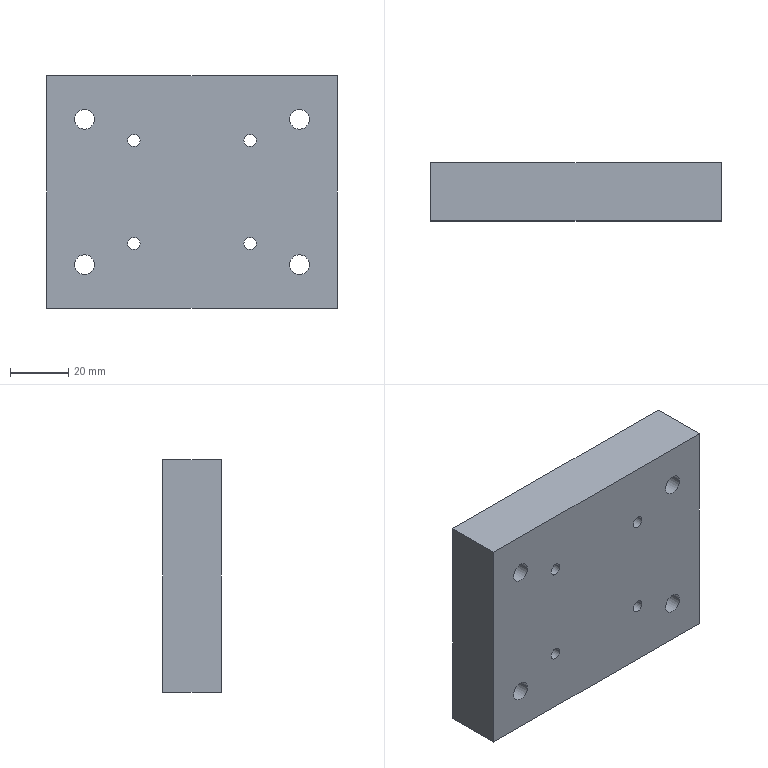Component | SolidWorks | RotaryCylinderBase-1 | 1 solid | 22 faces | box 100 x 20 x 80 mm | volume 155986 mm3 | cylinder 16 | plane 6 | commonest cylinder face diameters 6.8 x8 4.2 x8
build123d program:
from build123d import *

# Parameters (mm, degrees)
SKETCH2_W           = 100
SKETCH2_H           = 80
BOSS_EXTRUDE1_DEPTH = 20
M5_TAPPED_HOLE1_D   = 4.2
M8_TAPPED_HOLE1_D   = 6.8


with BuildPart() as part:
    # Sketch2 → Boss-Extrude1 (new body)
    with BuildSketch(Plane.XY):
        with Locations((233.487, -347.329)):
            Rectangle(SKETCH2_W, SKETCH2_H)
    extrude(amount=BOSS_EXTRUDE1_DEPTH)

    # M5 Tapped Hole1 (through all)
    with Locations(Plane.XY.offset(20)):
        with Locations((213.487, -365.079), (253.487, -365.079), (253.487, -329.579), (213.487, -329.579)):
            Hole(M5_TAPPED_HOLE1_D / 2)

    # M8 Tapped Hole1 (through all)
    with Locations(Plane(origin=(196.487, -322.329, 20), x_dir=(1, 0, 0), z_dir=(0, 0, 1))):
        with Locations((0, 0), (0, -50), (74, -50), (74, 0)):
            Hole(M8_TAPPED_HOLE1_D / 2)


solid = part.part

# Placed as in the assembly
solid = solid.moved(Location((-565.183, -127.651, 692.796), (90, 0, 0)))
STEP:
#1=COLOUR_RGB('',0.7922,0.8196,0.9333);
#2=FILL_AREA_STYLE_COLOUR('',#1);
#3=FILL_AREA_STYLE('',(#2));
#4=SURFACE_STYLE_FILL_AREA(#3);
#5=SURFACE_SIDE_STYLE('',(#4));
#6=SURFACE_STYLE_USAGE(.BOTH.,#5);
#7=PRESENTATION_STYLE_ASSIGNMENT((#6));
#8=CARTESIAN_POINT('',(-14.649,-5.813,12.617));
#9=VERTEX_POINT('',#8);
#10=CARTESIAN_POINT('',(-14.382,-5.813,12.617));
#11=VERTEX_POINT('',#10);
#12=CARTESIAN_POINT('',(-14.516,-5.813,12.617));
#13=DIRECTION('',(0.,1.,0.));
#14=DIRECTION('',(1.,0.,0.));
#15=AXIS2_PLACEMENT_3D('',#12,#13,#14);
#16=CIRCLE('',#15,0.1339);
#17=EDGE_CURVE('',#9,#11,#16,.T.);
#18=ORIENTED_EDGE('',*,*,#17,.F.);
#19=CARTESIAN_POINT('',(-14.649,-5.026,12.617));
#20=VERTEX_POINT('',#19);
#21=CARTESIAN_POINT('',(-14.649,-5.026,12.617));
#22=DIRECTION('',(0.,1.,0.));
#23=VECTOR('',#22,39.37);
#24=LINE('',#21,#23);
#25=EDGE_CURVE('',#9,#20,#24,.T.);
#26=ORIENTED_EDGE('',*,*,#25,.T.);
#27=CARTESIAN_POINT('',(-14.382,-5.026,12.617));
#28=VERTEX_POINT('',#27);
#29=CARTESIAN_POINT('',(-14.516,-5.026,12.617));
#30=DIRECTION('',(0.,1.,0.));
#31=DIRECTION('',(1.,0.,0.));
#32=AXIS2_PLACEMENT_3D('',#29,#30,#31);
#33=CIRCLE('',#32,0.1339);
#34=EDGE_CURVE('',#20,#28,#33,.T.);
#35=ORIENTED_EDGE('',*,*,#34,.T.);
#36=CARTESIAN_POINT('',(-14.382,-5.026,12.617));
#37=DIRECTION('',(0.,1.,0.));
#38=VECTOR('',#37,39.37);
#39=LINE('',#36,#38);
#40=EDGE_CURVE('',#11,#28,#39,.T.);
#41=ORIENTED_EDGE('',*,*,#40,.F.);
#42=EDGE_LOOP('',(#18,#26,#35,#41));
#43=FACE_OUTER_BOUND('',#42,.T.);
#44=CARTESIAN_POINT('',(-14.516,-5.026,12.617));
#45=DIRECTION('',(0.,1.,0.));
#46=DIRECTION('',(1.,0.,0.));
#47=AXIS2_PLACEMENT_3D('',#44,#45,#46);
#48=CYLINDRICAL_SURFACE('',#47,0.1339);
#49=ADVANCED_FACE('',(#43),#48,.F.);
#50=CARTESIAN_POINT('',(-14.649,-5.813,14.585));
#51=VERTEX_POINT('',#50);
#52=CARTESIAN_POINT('',(-14.382,-5.813,14.585));
#53=VERTEX_POINT('',#52);
#54=CARTESIAN_POINT('',(-14.516,-5.813,14.585));
#55=DIRECTION('',(0.,1.,0.));
#56=DIRECTION('',(1.,0.,0.));
#57=AXIS2_PLACEMENT_3D('',#54,#55,#56);
#58=CIRCLE('',#57,0.1339);
#59=EDGE_CURVE('',#51,#53,#58,.T.);
#60=ORIENTED_EDGE('',*,*,#59,.F.);
#61=CARTESIAN_POINT('',(-14.649,-5.026,14.585));
#62=VERTEX_POINT('',#61);
#63=CARTESIAN_POINT('',(-14.649,-5.026,14.585));
#64=DIRECTION('',(0.,1.,0.));
#65=VECTOR('',#64,39.37);
#66=LINE('',#63,#65);
#67=EDGE_CURVE('',#51,#62,#66,.T.);
#68=ORIENTED_EDGE('',*,*,#67,.T.);
#69=CARTESIAN_POINT('',(-14.382,-5.026,14.585));
#70=VERTEX_POINT('',#69);
#71=CARTESIAN_POINT('',(-14.516,-5.026,14.585));
#72=DIRECTION('',(0.,1.,0.));
#73=DIRECTION('',(1.,0.,0.));
#74=AXIS2_PLACEMENT_3D('',#71,#72,#73);
#75=CIRCLE('',#74,0.1339);
#76=EDGE_CURVE('',#62,#70,#75,.T.);
#77=ORIENTED_EDGE('',*,*,#76,.T.);
#78=CARTESIAN_POINT('',(-14.382,-5.026,14.585));
#79=DIRECTION('',(0.,1.,0.));
#80=VECTOR('',#79,39.37);
#81=LINE('',#78,#80);
#82=EDGE_CURVE('',#53,#70,#81,.T.);
#83=ORIENTED_EDGE('',*,*,#82,.F.);
#84=EDGE_LOOP('',(#60,#68,#77,#83));
#85=FACE_OUTER_BOUND('',#84,.T.);
#86=CARTESIAN_POINT('',(-14.516,-5.026,14.585));
#87=DIRECTION('',(0.,1.,0.));
#88=DIRECTION('',(1.,0.,0.));
#89=AXIS2_PLACEMENT_3D('',#86,#87,#88);
#90=CYLINDRICAL_SURFACE('',#89,0.1339);
#91=ADVANCED_FACE('',(#85),#90,.F.);
#92=CARTESIAN_POINT('',(-11.736,-5.813,14.585));
#93=VERTEX_POINT('',#92);
#94=CARTESIAN_POINT('',(-11.468,-5.813,14.585));
#95=VERTEX_POINT('',#94);
#96=CARTESIAN_POINT('',(-11.602,-5.813,14.585));
#97=DIRECTION('',(0.,1.,0.));
#98=DIRECTION('',(1.,0.,0.));
#99=AXIS2_PLACEMENT_3D('',#96,#97,#98);
#100=CIRCLE('',#99,0.1339);
#101=EDGE_CURVE('',#93,#95,#100,.T.);
#102=ORIENTED_EDGE('',*,*,#101,.F.);
#103=CARTESIAN_POINT('',(-11.736,-5.026,14.585));
#104=VERTEX_POINT('',#103);
#105=CARTESIAN_POINT('',(-11.736,-5.026,14.585));
#106=DIRECTION('',(0.,1.,0.));
#107=VECTOR('',#106,39.37);
#108=LINE('',#105,#107);
#109=EDGE_CURVE('',#93,#104,#108,.T.);
#110=ORIENTED_EDGE('',*,*,#109,.T.);
#111=CARTESIAN_POINT('',(-11.468,-5.026,14.585));
#112=VERTEX_POINT('',#111);
#113=CARTESIAN_POINT('',(-11.602,-5.026,14.585));
#114=DIRECTION('',(0.,1.,0.));
#115=DIRECTION('',(1.,0.,0.));
#116=AXIS2_PLACEMENT_3D('',#113,#114,#115);
#117=CIRCLE('',#116,0.1339);
#118=EDGE_CURVE('',#104,#112,#117,.T.);
#119=ORIENTED_EDGE('',*,*,#118,.T.);
#120=CARTESIAN_POINT('',(-11.468,-5.026,14.585));
#121=DIRECTION('',(0.,1.,0.));
#122=VECTOR('',#121,39.37);
#123=LINE('',#120,#122);
#124=EDGE_CURVE('',#95,#112,#123,.T.);
#125=ORIENTED_EDGE('',*,*,#124,.F.);
#126=EDGE_LOOP('',(#102,#110,#119,#125));
#127=FACE_OUTER_BOUND('',#126,.T.);
#128=CARTESIAN_POINT('',(-11.602,-5.026,14.585));
#129=DIRECTION('',(0.,1.,0.));
#130=DIRECTION('',(1.,0.,0.));
#131=AXIS2_PLACEMENT_3D('',#128,#129,#130);
#132=CYLINDRICAL_SURFACE('',#131,0.1339);
#133=ADVANCED_FACE('',(#127),#132,.F.);
#134=CARTESIAN_POINT('',(-11.736,-5.813,12.617));
#135=VERTEX_POINT('',#134);
#136=CARTESIAN_POINT('',(-11.468,-5.813,12.617));
#137=VERTEX_POINT('',#136);
#138=CARTESIAN_POINT('',(-11.602,-5.813,12.617));
#139=DIRECTION('',(0.,1.,0.));
#140=DIRECTION('',(1.,0.,0.));
#141=AXIS2_PLACEMENT_3D('',#138,#139,#140);
#142=CIRCLE('',#141,0.1339);
#143=EDGE_CURVE('',#135,#137,#142,.T.);
#144=ORIENTED_EDGE('',*,*,#143,.F.);
#145=CARTESIAN_POINT('',(-11.736,-5.026,12.617));
#146=VERTEX_POINT('',#145);
#147=CARTESIAN_POINT('',(-11.736,-5.026,12.617));
#148=DIRECTION('',(0.,1.,0.));
#149=VECTOR('',#148,39.37);
#150=LINE('',#147,#149);
#151=EDGE_CURVE('',#135,#146,#150,.T.);
#152=ORIENTED_EDGE('',*,*,#151,.T.);
#153=CARTESIAN_POINT('',(-11.468,-5.026,12.617));
#154=VERTEX_POINT('',#153);
#155=CARTESIAN_POINT('',(-11.602,-5.026,12.617));
#156=DIRECTION('',(0.,1.,0.));
#157=DIRECTION('',(1.,0.,0.));
#158=AXIS2_PLACEMENT_3D('',#155,#156,#157);
#159=CIRCLE('',#158,0.1339);
#160=EDGE_CURVE('',#146,#154,#159,.T.);
#161=ORIENTED_EDGE('',*,*,#160,.T.);
#162=CARTESIAN_POINT('',(-11.468,-5.026,12.617));
#163=DIRECTION('',(0.,1.,0.));
#164=VECTOR('',#163,39.37);
#165=LINE('',#162,#164);
#166=EDGE_CURVE('',#137,#154,#165,.T.);
#167=ORIENTED_EDGE('',*,*,#166,.F.);
#168=EDGE_LOOP('',(#144,#152,#161,#167));
#169=FACE_OUTER_BOUND('',#168,.T.);
#170=CARTESIAN_POINT('',(-11.602,-5.026,12.617));
#171=DIRECTION('',(0.,1.,0.));
#172=DIRECTION('',(1.,0.,0.));
#173=AXIS2_PLACEMENT_3D('',#170,#171,#172);
#174=CYLINDRICAL_SURFACE('',#173,0.1339);
#175=ADVANCED_FACE('',(#169),#174,.F.);
#176=CARTESIAN_POINT('',(-13.929,-5.813,14.3));
#177=VERTEX_POINT('',#176);
#178=CARTESIAN_POINT('',(-13.764,-5.813,14.3));
#179=VERTEX_POINT('',#178);
#180=CARTESIAN_POINT('',(-13.846,-5.813,14.3));
#181=DIRECTION('',(0.,1.,0.));
#182=DIRECTION('',(1.,0.,0.));
#183=AXIS2_PLACEMENT_3D('',#180,#181,#182);
#184=CIRCLE('',#183,0.08268);
#185=EDGE_CURVE('',#177,#179,#184,.T.);
#186=ORIENTED_EDGE('',*,*,#185,.F.);
#187=CARTESIAN_POINT('',(-13.929,-5.026,14.3));
#188=VERTEX_POINT('',#187);
#189=CARTESIAN_POINT('',(-13.929,-5.026,14.3));
#190=DIRECTION('',(0.,1.,0.));
#191=VECTOR('',#190,39.37);
#192=LINE('',#189,#191);
#193=EDGE_CURVE('',#177,#188,#192,.T.);
#194=ORIENTED_EDGE('',*,*,#193,.T.);
#195=CARTESIAN_POINT('',(-13.764,-5.026,14.3));
#196=VERTEX_POINT('',#195);
#197=CARTESIAN_POINT('',(-13.846,-5.026,14.3));
#198=DIRECTION('',(0.,1.,0.));
#199=DIRECTION('',(1.,0.,0.));
#200=AXIS2_PLACEMENT_3D('',#197,#198,#199);
#201=CIRCLE('',#200,0.08268);
#202=EDGE_CURVE('',#188,#196,#201,.T.);
#203=ORIENTED_EDGE('',*,*,#202,.T.);
#204=CARTESIAN_POINT('',(-13.764,-5.026,14.3));
#205=DIRECTION('',(0.,1.,0.));
#206=VECTOR('',#205,39.37);
#207=LINE('',#204,#206);
#208=EDGE_CURVE('',#179,#196,#207,.T.);
#209=ORIENTED_EDGE('',*,*,#208,.F.);
#210=EDGE_LOOP('',(#186,#194,#203,#209));
#211=FACE_OUTER_BOUND('',#210,.T.);
#212=CARTESIAN_POINT('',(-13.846,-5.026,14.3));
#213=DIRECTION('',(0.,1.,0.));
#214=DIRECTION('',(1.,0.,0.));
#215=AXIS2_PLACEMENT_3D('',#212,#213,#214);
#216=CYLINDRICAL_SURFACE('',#215,0.08268);
#217=ADVANCED_FACE('',(#211),#216,.F.);
#218=CARTESIAN_POINT('',(-12.354,-5.813,14.3));
#219=VERTEX_POINT('',#218);
#220=CARTESIAN_POINT('',(-12.189,-5.813,14.3));
#221=VERTEX_POINT('',#220);
#222=CARTESIAN_POINT('',(-12.271,-5.813,14.3));
#223=DIRECTION('',(0.,1.,0.));
#224=DIRECTION('',(1.,0.,0.));
#225=AXIS2_PLACEMENT_3D('',#222,#223,#224);
#226=CIRCLE('',#225,0.08268);
#227=EDGE_CURVE('',#219,#221,#226,.T.);
#228=ORIENTED_EDGE('',*,*,#227,.F.);
#229=CARTESIAN_POINT('',(-12.354,-5.026,14.3));
#230=VERTEX_POINT('',#229);
#231=CARTESIAN_POINT('',(-12.354,-5.026,14.3));
#232=DIRECTION('',(0.,1.,0.));
#233=VECTOR('',#232,39.37);
#234=LINE('',#231,#233);
#235=EDGE_CURVE('',#219,#230,#234,.T.);
#236=ORIENTED_EDGE('',*,*,#235,.T.);
#237=CARTESIAN_POINT('',(-12.189,-5.026,14.3));
#238=VERTEX_POINT('',#237);
#239=CARTESIAN_POINT('',(-12.271,-5.026,14.3));
#240=DIRECTION('',(0.,1.,0.));
#241=DIRECTION('',(1.,0.,0.));
#242=AXIS2_PLACEMENT_3D('',#239,#240,#241);
#243=CIRCLE('',#242,0.08268);
#244=EDGE_CURVE('',#230,#238,#243,.T.);
#245=ORIENTED_EDGE('',*,*,#244,.T.);
#246=CARTESIAN_POINT('',(-12.189,-5.026,14.3));
#247=DIRECTION('',(0.,1.,0.));
#248=VECTOR('',#247,39.37);
#249=LINE('',#246,#248);
#250=EDGE_CURVE('',#221,#238,#249,.T.);
#251=ORIENTED_EDGE('',*,*,#250,.F.);
#252=EDGE_LOOP('',(#228,#236,#245,#251));
#253=FACE_OUTER_BOUND('',#252,.T.);
#254=CARTESIAN_POINT('',(-12.271,-5.026,14.3));
#255=DIRECTION('',(0.,1.,0.));
#256=DIRECTION('',(1.,0.,0.));
#257=AXIS2_PLACEMENT_3D('',#254,#255,#256);
#258=CYLINDRICAL_SURFACE('',#257,0.08268);
#259=ADVANCED_FACE('',(#253),#258,.F.);
#260=CARTESIAN_POINT('',(-12.354,-5.813,12.902));
#261=VERTEX_POINT('',#260);
#262=CARTESIAN_POINT('',(-12.189,-5.813,12.902));
#263=VERTEX_POINT('',#262);
#264=CARTESIAN_POINT('',(-12.271,-5.813,12.902));
#265=DIRECTION('',(0.,1.,0.));
#266=DIRECTION('',(1.,0.,0.));
#267=AXIS2_PLACEMENT_3D('',#264,#265,#266);
#268=CIRCLE('',#267,0.08268);
#269=EDGE_CURVE('',#261,#263,#268,.T.);
#270=ORIENTED_EDGE('',*,*,#269,.F.);
#271=CARTESIAN_POINT('',(-12.354,-5.026,12.902));
#272=VERTEX_POINT('',#271);
#273=CARTESIAN_POINT('',(-12.354,-5.026,12.902));
#274=DIRECTION('',(0.,1.,0.));
#275=VECTOR('',#274,39.37);
#276=LINE('',#273,#275);
#277=EDGE_CURVE('',#261,#272,#276,.T.);
#278=ORIENTED_EDGE('',*,*,#277,.T.);
#279=CARTESIAN_POINT('',(-12.189,-5.026,12.902));
#280=VERTEX_POINT('',#279);
#281=CARTESIAN_POINT('',(-12.271,-5.026,12.902));
#282=DIRECTION('',(0.,1.,0.));
#283=DIRECTION('',(1.,0.,0.));
#284=AXIS2_PLACEMENT_3D('',#281,#282,#283);
#285=CIRCLE('',#284,0.08268);
#286=EDGE_CURVE('',#272,#280,#285,.T.);
#287=ORIENTED_EDGE('',*,*,#286,.T.);
#288=CARTESIAN_POINT('',(-12.189,-5.026,12.902));
#289=DIRECTION('',(0.,1.,0.));
#290=VECTOR('',#289,39.37);
#291=LINE('',#288,#290);
#292=EDGE_CURVE('',#263,#280,#291,.T.);
#293=ORIENTED_EDGE('',*,*,#292,.F.);
#294=EDGE_LOOP('',(#270,#278,#287,#293));
#295=FACE_OUTER_BOUND('',#294,.T.);
#296=CARTESIAN_POINT('',(-12.271,-5.026,12.902));
#297=DIRECTION('',(0.,1.,0.));
#298=DIRECTION('',(1.,0.,0.));
#299=AXIS2_PLACEMENT_3D('',#296,#297,#298);
#300=CYLINDRICAL_SURFACE('',#299,0.08268);
#301=ADVANCED_FACE('',(#295),#300,.F.);
#302=CARTESIAN_POINT('',(-13.929,-5.813,12.902));
#303=VERTEX_POINT('',#302);
#304=CARTESIAN_POINT('',(-13.764,-5.813,12.902));
#305=VERTEX_POINT('',#304);
#306=CARTESIAN_POINT('',(-13.846,-5.813,12.902));
#307=DIRECTION('',(0.,1.,0.));
#308=DIRECTION('',(1.,0.,0.));
#309=AXIS2_PLACEMENT_3D('',#306,#307,#308);
#310=CIRCLE('',#309,0.08268);
#311=EDGE_CURVE('',#303,#305,#310,.T.);
#312=ORIENTED_EDGE('',*,*,#311,.F.);
#313=CARTESIAN_POINT('',(-13.929,-5.026,12.902));
#314=VERTEX_POINT('',#313);
#315=CARTESIAN_POINT('',(-13.929,-5.026,12.902));
#316=DIRECTION('',(0.,1.,0.));
#317=VECTOR('',#316,39.37);
#318=LINE('',#315,#317);
#319=EDGE_CURVE('',#303,#314,#318,.T.);
#320=ORIENTED_EDGE('',*,*,#319,.T.);
#321=CARTESIAN_POINT('',(-13.764,-5.026,12.902));
#322=VERTEX_POINT('',#321);
#323=CARTESIAN_POINT('',(-13.846,-5.026,12.902));
#324=DIRECTION('',(0.,1.,0.));
#325=DIRECTION('',(1.,0.,0.));
#326=AXIS2_PLACEMENT_3D('',#323,#324,#325);
#327=CIRCLE('',#326,0.08268);
#328=EDGE_CURVE('',#314,#322,#327,.T.);
#329=ORIENTED_EDGE('',*,*,#328,.T.);
#330=CARTESIAN_POINT('',(-13.764,-5.026,12.902));
#331=DIRECTION('',(0.,1.,0.));
#332=VECTOR('',#331,39.37);
#333=LINE('',#330,#332);
#334=EDGE_CURVE('',#305,#322,#333,.T.);
#335=ORIENTED_EDGE('',*,*,#334,.F.);
#336=EDGE_LOOP('',(#312,#320,#329,#335));
#337=FACE_OUTER_BOUND('',#336,.T.);
#338=CARTESIAN_POINT('',(-13.846,-5.026,12.902));
#339=DIRECTION('',(0.,1.,0.));
#340=DIRECTION('',(1.,0.,0.));
#341=AXIS2_PLACEMENT_3D('',#338,#339,#340);
#342=CYLINDRICAL_SURFACE('',#341,0.08268);
#343=ADVANCED_FACE('',(#337),#342,.F.);
#344=CARTESIAN_POINT('',(-15.027,-5.813,12.026));
#345=VERTEX_POINT('',#344);
#346=CARTESIAN_POINT('',(-15.027,-5.813,15.176));
#347=VERTEX_POINT('',#346);
#348=CARTESIAN_POINT('',(-15.027,-5.813,12.026));
#349=DIRECTION('',(0.,-0.,1.));
#350=VECTOR('',#349,39.37);
#351=LINE('',#348,#350);
#352=EDGE_CURVE('',#345,#347,#351,.T.);
#353=ORIENTED_EDGE('',*,*,#352,.T.);
#354=CARTESIAN_POINT('',(-15.027,-5.026,15.176));
#355=VERTEX_POINT('',#354);
#356=CARTESIAN_POINT('',(-15.027,-5.026,15.176));
#357=DIRECTION('',(0.,-1.,-0.));
#358=VECTOR('',#357,39.37);
#359=LINE('',#356,#358);
#360=EDGE_CURVE('',#355,#347,#359,.T.);
#361=ORIENTED_EDGE('',*,*,#360,.F.);
#362=CARTESIAN_POINT('',(-15.027,-5.026,12.026));
#363=VERTEX_POINT('',#362);
#364=CARTESIAN_POINT('',(-15.027,-5.026,12.026));
#365=DIRECTION('',(0.,-0.,1.));
#366=VECTOR('',#365,39.37);
#367=LINE('',#364,#366);
#368=EDGE_CURVE('',#363,#355,#367,.T.);
#369=ORIENTED_EDGE('',*,*,#368,.F.);
#370=CARTESIAN_POINT('',(-15.027,-5.026,12.026));
#371=DIRECTION('',(0.,-1.,-0.));
#372=VECTOR('',#371,39.37);
#373=LINE('',#370,#372);
#374=EDGE_CURVE('',#363,#345,#373,.T.);
#375=ORIENTED_EDGE('',*,*,#374,.T.);
#376=EDGE_LOOP('',(#353,#361,#369,#375));
#377=FACE_OUTER_BOUND('',#376,.T.);
#378=CARTESIAN_POINT('',(-15.027,-5.026,12.026));
#379=DIRECTION('',(1.,0.,0.));
#380=DIRECTION('',(0.,-1.,-0.));
#381=AXIS2_PLACEMENT_3D('',#378,#379,#380);
#382=PLANE('',#381);
#383=ADVANCED_FACE('',(#377),#382,.F.);
#384=CARTESIAN_POINT('',(-11.09,-5.813,15.176));
#385=VERTEX_POINT('',#384);
#386=CARTESIAN_POINT('',(-15.027,-5.813,15.176));
#387=DIRECTION('',(1.,0.,0.));
#388=VECTOR('',#387,39.37);
#389=LINE('',#386,#388);
#390=EDGE_CURVE('',#347,#385,#389,.T.);
#391=ORIENTED_EDGE('',*,*,#390,.T.);
#392=CARTESIAN_POINT('',(-11.09,-5.026,15.176));
#393=VERTEX_POINT('',#392);
#394=CARTESIAN_POINT('',(-11.09,-5.026,15.176));
#395=DIRECTION('',(0.,-1.,-0.));
#396=VECTOR('',#395,39.37);
#397=LINE('',#394,#396);
#398=EDGE_CURVE('',#393,#385,#397,.T.);
#399=ORIENTED_EDGE('',*,*,#398,.F.);
#400=CARTESIAN_POINT('',(-15.027,-5.026,15.176));
#401=DIRECTION('',(1.,0.,0.));
#402=VECTOR('',#401,39.37);
#403=LINE('',#400,#402);
#404=EDGE_CURVE('',#355,#393,#403,.T.);
#405=ORIENTED_EDGE('',*,*,#404,.F.);
#406=ORIENTED_EDGE('',*,*,#360,.T.);
#407=EDGE_LOOP('',(#391,#399,#405,#406));
#408=FACE_OUTER_BOUND('',#407,.T.);
#409=CARTESIAN_POINT('',(-15.027,-5.026,15.176));
#410=DIRECTION('',(0.,0.,-1.));
#411=DIRECTION('',(0.,1.,0.));
#412=AXIS2_PLACEMENT_3D('',#409,#410,#411);
#413=PLANE('',#412);
#414=ADVANCED_FACE('',(#408),#413,.F.);
#415=CARTESIAN_POINT('',(-11.09,-5.813,12.026));
#416=VERTEX_POINT('',#415);
#417=CARTESIAN_POINT('',(-11.09,-5.813,12.026));
#418=DIRECTION('',(0.,0.,-1.));
#419=VECTOR('',#418,39.37);
#420=LINE('',#417,#419);
#421=EDGE_CURVE('',#385,#416,#420,.T.);
#422=ORIENTED_EDGE('',*,*,#421,.T.);
#423=CARTESIAN_POINT('',(-11.09,-5.026,12.026));
#424=VERTEX_POINT('',#423);
#425=CARTESIAN_POINT('',(-11.09,-5.026,12.026));
#426=DIRECTION('',(0.,-1.,-0.));
#427=VECTOR('',#426,39.37);
#428=LINE('',#425,#427);
#429=EDGE_CURVE('',#424,#416,#428,.T.);
#430=ORIENTED_EDGE('',*,*,#429,.F.);
#431=CARTESIAN_POINT('',(-11.09,-5.026,12.026));
#432=DIRECTION('',(0.,0.,-1.));
#433=VECTOR('',#432,39.37);
#434=LINE('',#431,#433);
#435=EDGE_CURVE('',#393,#424,#434,.T.);
#436=ORIENTED_EDGE('',*,*,#435,.F.);
#437=ORIENTED_EDGE('',*,*,#398,.T.);
#438=EDGE_LOOP('',(#422,#430,#436,#437));
#439=FACE_OUTER_BOUND('',#438,.T.);
#440=CARTESIAN_POINT('',(-11.09,-5.026,12.026));
#441=DIRECTION('',(-1.,0.,0.));
#442=DIRECTION('',(0.,1.,0.));
#443=AXIS2_PLACEMENT_3D('',#440,#441,#442);
#444=PLANE('',#443);
#445=ADVANCED_FACE('',(#439),#444,.F.);
#446=CARTESIAN_POINT('',(-15.027,-5.813,12.026));
#447=DIRECTION('',(-1.,0.,0.));
#448=VECTOR('',#447,39.37);
#449=LINE('',#446,#448);
#450=EDGE_CURVE('',#416,#345,#449,.T.);
#451=ORIENTED_EDGE('',*,*,#450,.T.);
#452=ORIENTED_EDGE('',*,*,#374,.F.);
#453=CARTESIAN_POINT('',(-15.027,-5.026,12.026));
#454=DIRECTION('',(-1.,0.,0.));
#455=VECTOR('',#454,39.37);
#456=LINE('',#453,#455);
#457=EDGE_CURVE('',#424,#363,#456,.T.);
#458=ORIENTED_EDGE('',*,*,#457,.F.);
#459=ORIENTED_EDGE('',*,*,#429,.T.);
#460=EDGE_LOOP('',(#451,#452,#458,#459));
#461=FACE_OUTER_BOUND('',#460,.T.);
#462=CARTESIAN_POINT('',(-15.027,-5.026,12.026));
#463=DIRECTION('',(0.,-0.,1.));
#464=DIRECTION('',(0.,-1.,-0.));
#465=AXIS2_PLACEMENT_3D('',#462,#463,#464);
#466=PLANE('',#465);
#467=ADVANCED_FACE('',(#461),#466,.F.);
#468=CARTESIAN_POINT('',(-14.516,-5.026,12.617));
#469=DIRECTION('',(0.,1.,0.));
#470=DIRECTION('',(1.,0.,0.));
#471=AXIS2_PLACEMENT_3D('',#468,#469,#470);
#472=CIRCLE('',#471,0.1339);
#473=EDGE_CURVE('',#28,#20,#472,.T.);
#474=ORIENTED_EDGE('',*,*,#473,.F.);
#475=ORIENTED_EDGE('',*,*,#34,.F.);
#476=EDGE_LOOP('',(#474,#475));
#477=FACE_BOUND('',#476,.T.);
#478=CARTESIAN_POINT('',(-14.516,-5.026,14.585));
#479=DIRECTION('',(0.,1.,0.));
#480=DIRECTION('',(1.,0.,0.));
#481=AXIS2_PLACEMENT_3D('',#478,#479,#480);
#482=CIRCLE('',#481,0.1339);
#483=EDGE_CURVE('',#70,#62,#482,.T.);
#484=ORIENTED_EDGE('',*,*,#483,.F.);
#485=ORIENTED_EDGE('',*,*,#76,.F.);
#486=EDGE_LOOP('',(#484,#485));
#487=FACE_BOUND('',#486,.T.);
#488=CARTESIAN_POINT('',(-11.602,-5.026,14.585));
#489=DIRECTION('',(0.,1.,0.));
#490=DIRECTION('',(1.,0.,0.));
#491=AXIS2_PLACEMENT_3D('',#488,#489,#490);
#492=CIRCLE('',#491,0.1339);
#493=EDGE_CURVE('',#112,#104,#492,.T.);
#494=ORIENTED_EDGE('',*,*,#493,.F.);
#495=ORIENTED_EDGE('',*,*,#118,.F.);
#496=EDGE_LOOP('',(#494,#495));
#497=FACE_BOUND('',#496,.T.);
#498=CARTESIAN_POINT('',(-11.602,-5.026,12.617));
#499=DIRECTION('',(0.,1.,0.));
#500=DIRECTION('',(1.,0.,0.));
#501=AXIS2_PLACEMENT_3D('',#498,#499,#500);
#502=CIRCLE('',#501,0.1339);
#503=EDGE_CURVE('',#154,#146,#502,.T.);
#504=ORIENTED_EDGE('',*,*,#503,.F.);
#505=ORIENTED_EDGE('',*,*,#160,.F.);
#506=EDGE_LOOP('',(#504,#505));
#507=FACE_BOUND('',#506,.T.);
#508=CARTESIAN_POINT('',(-13.846,-5.026,14.3));
#509=DIRECTION('',(0.,1.,0.));
#510=DIRECTION('',(1.,0.,0.));
#511=AXIS2_PLACEMENT_3D('',#508,#509,#510);
#512=CIRCLE('',#511,0.08268);
#513=EDGE_CURVE('',#196,#188,#512,.T.);
#514=ORIENTED_EDGE('',*,*,#513,.F.);
#515=ORIENTED_EDGE('',*,*,#202,.F.);
#516=EDGE_LOOP('',(#514,#515));
#517=FACE_BOUND('',#516,.T.);
#518=CARTESIAN_POINT('',(-12.271,-5.026,14.3));
#519=DIRECTION('',(0.,1.,0.));
#520=DIRECTION('',(1.,0.,0.));
#521=AXIS2_PLACEMENT_3D('',#518,#519,#520);
#522=CIRCLE('',#521,0.08268);
#523=EDGE_CURVE('',#238,#230,#522,.T.);
#524=ORIENTED_EDGE('',*,*,#523,.F.);
#525=ORIENTED_EDGE('',*,*,#244,.F.);
#526=EDGE_LOOP('',(#524,#525));
#527=FACE_BOUND('',#526,.T.);
#528=CARTESIAN_POINT('',(-12.271,-5.026,12.902));
#529=DIRECTION('',(0.,1.,0.));
#530=DIRECTION('',(1.,0.,0.));
#531=AXIS2_PLACEMENT_3D('',#528,#529,#530);
#532=CIRCLE('',#531,0.08268);
#533=EDGE_CURVE('',#280,#272,#532,.T.);
#534=ORIENTED_EDGE('',*,*,#533,.F.);
#535=ORIENTED_EDGE('',*,*,#286,.F.);
#536=EDGE_LOOP('',(#534,#535));
#537=FACE_BOUND('',#536,.T.);
#538=CARTESIAN_POINT('',(-13.846,-5.026,12.902));
#539=DIRECTION('',(0.,1.,0.));
#540=DIRECTION('',(1.,0.,0.));
#541=AXIS2_PLACEMENT_3D('',#538,#539,#540);
#542=CIRCLE('',#541,0.08268);
#543=EDGE_CURVE('',#322,#314,#542,.T.);
#544=ORIENTED_EDGE('',*,*,#543,.F.);
#545=ORIENTED_EDGE('',*,*,#328,.F.);
#546=EDGE_LOOP('',(#544,#545));
#547=FACE_BOUND('',#546,.T.);
#548=ORIENTED_EDGE('',*,*,#368,.T.);
#549=ORIENTED_EDGE('',*,*,#404,.T.);
#550=ORIENTED_EDGE('',*,*,#435,.T.);
#551=ORIENTED_EDGE('',*,*,#457,.T.);
#552=EDGE_LOOP('',(#548,#549,#550,#551));
#553=FACE_OUTER_BOUND('',#552,.T.);
#554=CARTESIAN_POINT('',(-22.251,-5.026,-0.07327));
#555=DIRECTION('',(0.,1.,0.));
#556=DIRECTION('',(1.,0.,0.));
#557=AXIS2_PLACEMENT_3D('',#554,#555,#556);
#558=PLANE('',#557);
#559=ADVANCED_FACE('',(#477,#487,#497,#507,#517,#527,#537,#547,#553),#558,.T.);
#560=CARTESIAN_POINT('',(-14.516,-5.813,12.617));
#561=DIRECTION('',(0.,1.,0.));
#562=DIRECTION('',(1.,0.,0.));
#563=AXIS2_PLACEMENT_3D('',#560,#561,#562);
#564=CIRCLE('',#563,0.1339);
#565=EDGE_CURVE('',#11,#9,#564,.T.);
#566=ORIENTED_EDGE('',*,*,#565,.T.);
#567=ORIENTED_EDGE('',*,*,#17,.T.);
#568=EDGE_LOOP('',(#566,#567));
#569=FACE_BOUND('',#568,.T.);
#570=CARTESIAN_POINT('',(-14.516,-5.813,14.585));
#571=DIRECTION('',(0.,1.,0.));
#572=DIRECTION('',(1.,0.,0.));
#573=AXIS2_PLACEMENT_3D('',#570,#571,#572);
#574=CIRCLE('',#573,0.1339);
#575=EDGE_CURVE('',#53,#51,#574,.T.);
#576=ORIENTED_EDGE('',*,*,#575,.T.);
#577=ORIENTED_EDGE('',*,*,#59,.T.);
#578=EDGE_LOOP('',(#576,#577));
#579=FACE_BOUND('',#578,.T.);
#580=CARTESIAN_POINT('',(-11.602,-5.813,14.585));
#581=DIRECTION('',(0.,1.,0.));
#582=DIRECTION('',(1.,0.,0.));
#583=AXIS2_PLACEMENT_3D('',#580,#581,#582);
#584=CIRCLE('',#583,0.1339);
#585=EDGE_CURVE('',#95,#93,#584,.T.);
#586=ORIENTED_EDGE('',*,*,#585,.T.);
#587=ORIENTED_EDGE('',*,*,#101,.T.);
#588=EDGE_LOOP('',(#586,#587));
#589=FACE_BOUND('',#588,.T.);
#590=CARTESIAN_POINT('',(-11.602,-5.813,12.617));
#591=DIRECTION('',(0.,1.,0.));
#592=DIRECTION('',(1.,0.,0.));
#593=AXIS2_PLACEMENT_3D('',#590,#591,#592);
#594=CIRCLE('',#593,0.1339);
#595=EDGE_CURVE('',#137,#135,#594,.T.);
#596=ORIENTED_EDGE('',*,*,#595,.T.);
#597=ORIENTED_EDGE('',*,*,#143,.T.);
#598=EDGE_LOOP('',(#596,#597));
#599=FACE_BOUND('',#598,.T.);
#600=CARTESIAN_POINT('',(-13.846,-5.813,14.3));
#601=DIRECTION('',(0.,1.,0.));
#602=DIRECTION('',(1.,0.,0.));
#603=AXIS2_PLACEMENT_3D('',#600,#601,#602);
#604=CIRCLE('',#603,0.08268);
#605=EDGE_CURVE('',#179,#177,#604,.T.);
#606=ORIENTED_EDGE('',*,*,#605,.T.);
#607=ORIENTED_EDGE('',*,*,#185,.T.);
#608=EDGE_LOOP('',(#606,#607));
#609=FACE_BOUND('',#608,.T.);
#610=CARTESIAN_POINT('',(-12.271,-5.813,14.3));
#611=DIRECTION('',(0.,1.,0.));
#612=DIRECTION('',(1.,0.,0.));
#613=AXIS2_PLACEMENT_3D('',#610,#611,#612);
#614=CIRCLE('',#613,0.08268);
#615=EDGE_CURVE('',#221,#219,#614,.T.);
#616=ORIENTED_EDGE('',*,*,#615,.T.);
#617=ORIENTED_EDGE('',*,*,#227,.T.);
#618=EDGE_LOOP('',(#616,#617));
#619=FACE_BOUND('',#618,.T.);
#620=CARTESIAN_POINT('',(-12.271,-5.813,12.902));
#621=DIRECTION('',(0.,1.,0.));
#622=DIRECTION('',(1.,0.,0.));
#623=AXIS2_PLACEMENT_3D('',#620,#621,#622);
#624=CIRCLE('',#623,0.08268);
#625=EDGE_CURVE('',#263,#261,#624,.T.);
#626=ORIENTED_EDGE('',*,*,#625,.T.);
#627=ORIENTED_EDGE('',*,*,#269,.T.);
#628=EDGE_LOOP('',(#626,#627));
#629=FACE_BOUND('',#628,.T.);
#630=CARTESIAN_POINT('',(-13.846,-5.813,12.902));
#631=DIRECTION('',(0.,1.,0.));
#632=DIRECTION('',(1.,0.,0.));
#633=AXIS2_PLACEMENT_3D('',#630,#631,#632);
#634=CIRCLE('',#633,0.08268);
#635=EDGE_CURVE('',#305,#303,#634,.T.);
#636=ORIENTED_EDGE('',*,*,#635,.T.);
#637=ORIENTED_EDGE('',*,*,#311,.T.);
#638=EDGE_LOOP('',(#636,#637));
#639=FACE_BOUND('',#638,.T.);
#640=ORIENTED_EDGE('',*,*,#352,.F.);
#641=ORIENTED_EDGE('',*,*,#450,.F.);
#642=ORIENTED_EDGE('',*,*,#421,.F.);
#643=ORIENTED_EDGE('',*,*,#390,.F.);
#644=EDGE_LOOP('',(#640,#641,#642,#643));
#645=FACE_OUTER_BOUND('',#644,.T.);
#646=CARTESIAN_POINT('',(-22.251,-5.813,-0.07327));
#647=DIRECTION('',(0.,1.,0.));
#648=DIRECTION('',(1.,0.,0.));
#649=AXIS2_PLACEMENT_3D('',#646,#647,#648);
#650=PLANE('',#649);
#651=ADVANCED_FACE('',(#569,#579,#589,#599,#609,#619,#629,#639,#645),#650,.F.);
#652=ORIENTED_EDGE('',*,*,#319,.F.);
#653=ORIENTED_EDGE('',*,*,#635,.F.);
#654=ORIENTED_EDGE('',*,*,#334,.T.);
#655=ORIENTED_EDGE('',*,*,#543,.T.);
#656=EDGE_LOOP('',(#652,#653,#654,#655));
#657=FACE_OUTER_BOUND('',#656,.T.);
#658=CARTESIAN_POINT('',(-13.846,-5.026,12.902));
#659=DIRECTION('',(0.,1.,0.));
#660=DIRECTION('',(1.,0.,0.));
#661=AXIS2_PLACEMENT_3D('',#658,#659,#660);
#662=CYLINDRICAL_SURFACE('',#661,0.08268);
#663=ADVANCED_FACE('',(#657),#662,.F.);
#664=ORIENTED_EDGE('',*,*,#277,.F.);
#665=ORIENTED_EDGE('',*,*,#625,.F.);
#666=ORIENTED_EDGE('',*,*,#292,.T.);
#667=ORIENTED_EDGE('',*,*,#533,.T.);
#668=EDGE_LOOP('',(#664,#665,#666,#667));
#669=FACE_OUTER_BOUND('',#668,.T.);
#670=CARTESIAN_POINT('',(-12.271,-5.026,12.902));
#671=DIRECTION('',(0.,1.,0.));
#672=DIRECTION('',(1.,0.,0.));
#673=AXIS2_PLACEMENT_3D('',#670,#671,#672);
#674=CYLINDRICAL_SURFACE('',#673,0.08268);
#675=ADVANCED_FACE('',(#669),#674,.F.);
#676=ORIENTED_EDGE('',*,*,#235,.F.);
#677=ORIENTED_EDGE('',*,*,#615,.F.);
#678=ORIENTED_EDGE('',*,*,#250,.T.);
#679=ORIENTED_EDGE('',*,*,#523,.T.);
#680=EDGE_LOOP('',(#676,#677,#678,#679));
#681=FACE_OUTER_BOUND('',#680,.T.);
#682=CARTESIAN_POINT('',(-12.271,-5.026,14.3));
#683=DIRECTION('',(0.,1.,0.));
#684=DIRECTION('',(1.,0.,0.));
#685=AXIS2_PLACEMENT_3D('',#682,#683,#684);
#686=CYLINDRICAL_SURFACE('',#685,0.08268);
#687=ADVANCED_FACE('',(#681),#686,.F.);
#688=ORIENTED_EDGE('',*,*,#193,.F.);
#689=ORIENTED_EDGE('',*,*,#605,.F.);
#690=ORIENTED_EDGE('',*,*,#208,.T.);
#691=ORIENTED_EDGE('',*,*,#513,.T.);
#692=EDGE_LOOP('',(#688,#689,#690,#691));
#693=FACE_OUTER_BOUND('',#692,.T.);
#694=CARTESIAN_POINT('',(-13.846,-5.026,14.3));
#695=DIRECTION('',(0.,1.,0.));
#696=DIRECTION('',(1.,0.,0.));
#697=AXIS2_PLACEMENT_3D('',#694,#695,#696);
#698=CYLINDRICAL_SURFACE('',#697,0.08268);
#699=ADVANCED_FACE('',(#693),#698,.F.);
#700=ORIENTED_EDGE('',*,*,#151,.F.);
#701=ORIENTED_EDGE('',*,*,#595,.F.);
#702=ORIENTED_EDGE('',*,*,#166,.T.);
#703=ORIENTED_EDGE('',*,*,#503,.T.);
#704=EDGE_LOOP('',(#700,#701,#702,#703));
#705=FACE_OUTER_BOUND('',#704,.T.);
#706=CARTESIAN_POINT('',(-11.602,-5.026,12.617));
#707=DIRECTION('',(0.,1.,0.));
#708=DIRECTION('',(1.,0.,0.));
#709=AXIS2_PLACEMENT_3D('',#706,#707,#708);
#710=CYLINDRICAL_SURFACE('',#709,0.1339);
#711=ADVANCED_FACE('',(#705),#710,.F.);
#712=ORIENTED_EDGE('',*,*,#109,.F.);
#713=ORIENTED_EDGE('',*,*,#585,.F.);
#714=ORIENTED_EDGE('',*,*,#124,.T.);
#715=ORIENTED_EDGE('',*,*,#493,.T.);
#716=EDGE_LOOP('',(#712,#713,#714,#715));
#717=FACE_OUTER_BOUND('',#716,.T.);
#718=CARTESIAN_POINT('',(-11.602,-5.026,14.585));
#719=DIRECTION('',(0.,1.,0.));
#720=DIRECTION('',(1.,0.,0.));
#721=AXIS2_PLACEMENT_3D('',#718,#719,#720);
#722=CYLINDRICAL_SURFACE('',#721,0.1339);
#723=ADVANCED_FACE('',(#717),#722,.F.);
#724=ORIENTED_EDGE('',*,*,#67,.F.);
#725=ORIENTED_EDGE('',*,*,#575,.F.);
#726=ORIENTED_EDGE('',*,*,#82,.T.);
#727=ORIENTED_EDGE('',*,*,#483,.T.);
#728=EDGE_LOOP('',(#724,#725,#726,#727));
#729=FACE_OUTER_BOUND('',#728,.T.);
#730=CARTESIAN_POINT('',(-14.516,-5.026,14.585));
#731=DIRECTION('',(0.,1.,0.));
#732=DIRECTION('',(1.,0.,0.));
#733=AXIS2_PLACEMENT_3D('',#730,#731,#732);
#734=CYLINDRICAL_SURFACE('',#733,0.1339);
#735=ADVANCED_FACE('',(#729),#734,.F.);
#736=ORIENTED_EDGE('',*,*,#25,.F.);
#737=ORIENTED_EDGE('',*,*,#565,.F.);
#738=ORIENTED_EDGE('',*,*,#40,.T.);
#739=ORIENTED_EDGE('',*,*,#473,.T.);
#740=EDGE_LOOP('',(#736,#737,#738,#739));
#741=FACE_OUTER_BOUND('',#740,.T.);
#742=CARTESIAN_POINT('',(-14.516,-5.026,12.617));
#743=DIRECTION('',(0.,1.,0.));
#744=DIRECTION('',(1.,0.,0.));
#745=AXIS2_PLACEMENT_3D('',#742,#743,#744);
#746=CYLINDRICAL_SURFACE('',#745,0.1339);
#747=ADVANCED_FACE('',(#741),#746,.F.);
#748=CLOSED_SHELL('',(#49,#91,#133,#175,#217,#259,#301,#343,#383,#414,#445,#467,#559,#651,#663,#675,#687,#699,#711,#723,#735,#747));
#749=MANIFOLD_SOLID_BREP('',#748);
#750=STYLED_ITEM('',(#7),#749);
#751=PRESENTATION_LAYER_ASSIGNMENT('','',(#750));
#752=CARTESIAN_POINT('',(0.,0.,0.));
#753=DIRECTION('',(0.,0.,1.));
#754=DIRECTION('',(1.,0.,0.));
#755=AXIS2_PLACEMENT_3D('',#752,#753,#754);
#756=(LENGTH_UNIT()NAMED_UNIT(*)SI_UNIT($,.METRE.));
#757=LENGTH_MEASURE_WITH_UNIT(LENGTH_MEASURE(0.0254),#756);
#758=DIMENSIONAL_EXPONENTS(1.,0.,0.,0.,0.,0.,0.);
#759=(CONVERSION_BASED_UNIT('',#757)LENGTH_UNIT()NAMED_UNIT(#758));
#760=UNCERTAINTY_MEASURE_WITH_UNIT(LENGTH_MEASURE(0.00001),#759,'','');
#761=(NAMED_UNIT(*)PLANE_ANGLE_UNIT()SI_UNIT($,.RADIAN.));
#762=(NAMED_UNIT(*)SI_UNIT($,.STERADIAN.)SOLID_ANGLE_UNIT());
#763=(GEOMETRIC_REPRESENTATION_CONTEXT(3)GLOBAL_UNCERTAINTY_ASSIGNED_CONTEXT((#760))GLOBAL_UNIT_ASSIGNED_CONTEXT((#759,#761,#762))REPRESENTATION_CONTEXT('',''));
#764=ADVANCED_BREP_SHAPE_REPRESENTATION('',(#749,#755),#763);
#765=(LENGTH_UNIT()NAMED_UNIT(*)SI_UNIT($,.METRE.));
#766=LENGTH_MEASURE_WITH_UNIT(LENGTH_MEASURE(0.0254),#765);
#767=DIMENSIONAL_EXPONENTS(1.,0.,0.,0.,0.,0.,0.);
#768=(CONVERSION_BASED_UNIT('',#766)LENGTH_UNIT()NAMED_UNIT(#767));
#769=UNCERTAINTY_MEASURE_WITH_UNIT(LENGTH_MEASURE(0.00001),#768,'','');
#770=(NAMED_UNIT(*)PLANE_ANGLE_UNIT()SI_UNIT($,.RADIAN.));
#771=(NAMED_UNIT(*)SI_UNIT($,.STERADIAN.)SOLID_ANGLE_UNIT());
#772=(GEOMETRIC_REPRESENTATION_CONTEXT(3)GLOBAL_UNCERTAINTY_ASSIGNED_CONTEXT((#769))GLOBAL_UNIT_ASSIGNED_CONTEXT((#768,#770,#771))REPRESENTATION_CONTEXT('',''));
#773=MECHANICAL_DESIGN_GEOMETRIC_PRESENTATION_REPRESENTATION('',(#750),#772);